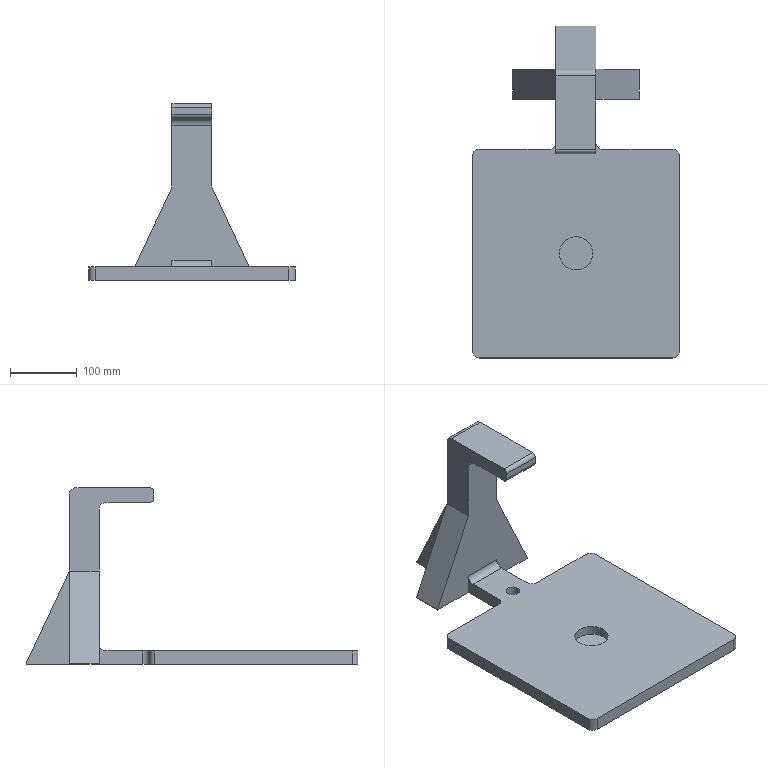Component | NX | ALTLIK | 1 solid | 44 faces | volume 3500120 mm3 | plane 29 | cylinder 15 | commonest cylinder face diameters 20 x12 12 x2 50 x1